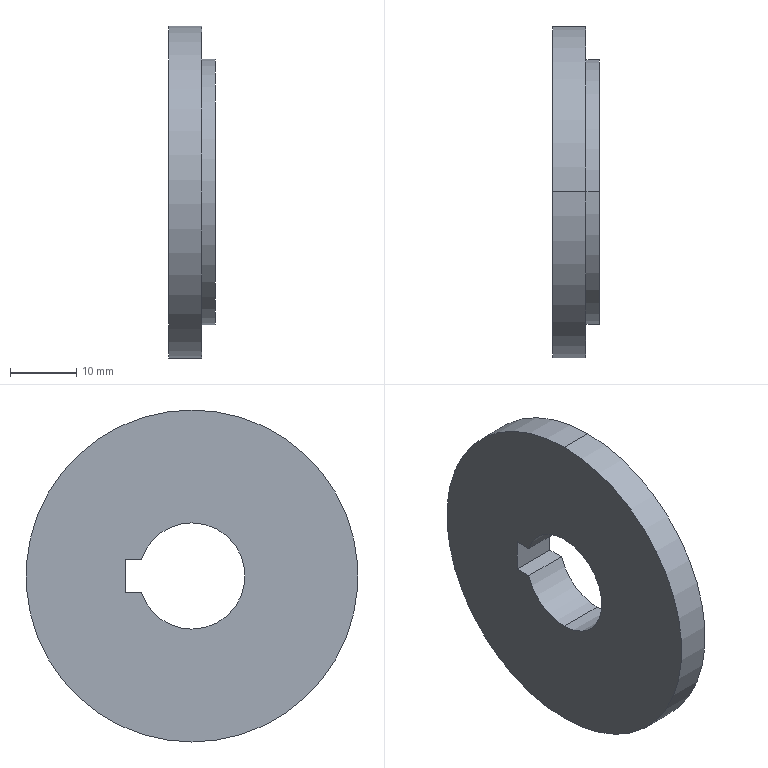Component | SolidWorks | MotorEndCover-1 | 1 solid | 13 faces | box 7 x 50 x 50 mm | volume 10847 mm3 | cylinder 7 | plane 6 | commonest cylinder face diameters 16 x3 50 x2 40 x2
build123d program:
from build123d import *

# Parameters (mm, degrees)
SKETCH2_R               = 20
BOSS_EXTRUDE1_DEPTH     = 2
SKETCH3_R               = 25
BOSS_EXTRUDE2_DEPTH     = 5
CUT_EXTRUDE1_DEPTH      = 37.042
CUT_EXTRUDE1_DEPTH_BACK = 37.042


with BuildPart() as part:
    # Sketch2 → Boss-Extrude1 (new body)
    with BuildSketch(Plane.XY):
        Circle(SKETCH2_R)
    extrude(amount=BOSS_EXTRUDE1_DEPTH)

    # Sketch3 → Boss-Extrude2 (add)
    with BuildSketch(Plane.XY.offset(2)):
        Circle(SKETCH3_R)
    extrude(amount=BOSS_EXTRUDE2_DEPTH)

    # Sketch4 → Cut-Extrude1 (cut, two sides: drawn at the far end of the back side and taken through both)
    with BuildSketch(Plane.XY.offset(7).offset(-CUT_EXTRUDE1_DEPTH_BACK)):
        with BuildLine():
            Line((-2.499, 7.6), (-2.499, 10.061))
            Line((-2.499, 10.061), (2.501, 10.061))
            Line((2.501, 10.061), (2.501, 7.599))
            ThreePointArc((2.501, 7.599), (-0.001053, -8), (-2.499, 7.6))
        make_face()
    extrude(amount=CUT_EXTRUDE1_DEPTH + CUT_EXTRUDE1_DEPTH_BACK, mode=Mode.SUBTRACT)


solid = part.part

# Placed as in the assembly
solid = solid.moved(Location((386.19, 335.1, 35), (0, -90, 0)))
STEP:
#1=COLOUR_RGB('',0.7922,0.8196,0.9333);
#2=FILL_AREA_STYLE_COLOUR('',#1);
#3=FILL_AREA_STYLE('',(#2));
#4=SURFACE_STYLE_FILL_AREA(#3);
#5=SURFACE_SIDE_STYLE('',(#4));
#6=SURFACE_STYLE_USAGE(.BOTH.,#5);
#7=PRESENTATION_STYLE_ASSIGNMENT((#6));
#8=CARTESIAN_POINT('',(15.204,13.193,1.063));
#9=VERTEX_POINT('',#8);
#10=CARTESIAN_POINT('',(15.204,13.193,1.693));
#11=VERTEX_POINT('',#10);
#12=CARTESIAN_POINT('',(15.204,13.193,1.378));
#13=DIRECTION('',(-1.,-0.,0.));
#14=DIRECTION('',(0.,-0.,1.));
#15=AXIS2_PLACEMENT_3D('',#12,#13,#14);
#16=CIRCLE('',#15,0.315);
#17=EDGE_CURVE('',#9,#11,#16,.T.);
#18=ORIENTED_EDGE('',*,*,#17,.F.);
#19=CARTESIAN_POINT('',(14.929,13.193,1.063));
#20=VERTEX_POINT('',#19);
#21=CARTESIAN_POINT('',(15.204,13.193,1.063));
#22=DIRECTION('',(-1.,-0.,0.));
#23=VECTOR('',#22,39.37);
#24=LINE('',#21,#23);
#25=EDGE_CURVE('',#9,#20,#24,.T.);
#26=ORIENTED_EDGE('',*,*,#25,.T.);
#27=CARTESIAN_POINT('',(14.929,13.193,1.693));
#28=VERTEX_POINT('',#27);
#29=CARTESIAN_POINT('',(14.929,13.193,1.378));
#30=DIRECTION('',(-1.,-0.,0.));
#31=DIRECTION('',(0.,-0.,1.));
#32=AXIS2_PLACEMENT_3D('',#29,#30,#31);
#33=CIRCLE('',#32,0.315);
#34=EDGE_CURVE('',#20,#28,#33,.T.);
#35=ORIENTED_EDGE('',*,*,#34,.T.);
#36=CARTESIAN_POINT('',(15.204,13.193,1.693));
#37=DIRECTION('',(-1.,-0.,0.));
#38=VECTOR('',#37,39.37);
#39=LINE('',#36,#38);
#40=EDGE_CURVE('',#11,#28,#39,.T.);
#41=ORIENTED_EDGE('',*,*,#40,.F.);
#42=EDGE_LOOP('',(#18,#26,#35,#41));
#43=FACE_OUTER_BOUND('',#42,.T.);
#44=CARTESIAN_POINT('',(15.204,13.193,1.378));
#45=DIRECTION('',(-1.,-0.,0.));
#46=DIRECTION('',(0.,-0.,1.));
#47=AXIS2_PLACEMENT_3D('',#44,#45,#46);
#48=CYLINDRICAL_SURFACE('',#47,0.315);
#49=ADVANCED_FACE('',(#43),#48,.F.);
#50=CARTESIAN_POINT('',(15.204,13.492,1.476));
#51=VERTEX_POINT('',#50);
#52=CARTESIAN_POINT('',(15.204,13.193,1.378));
#53=DIRECTION('',(-1.,-0.,0.));
#54=DIRECTION('',(0.,-0.,1.));
#55=AXIS2_PLACEMENT_3D('',#52,#53,#54);
#56=CIRCLE('',#55,0.315);
#57=EDGE_CURVE('',#11,#51,#56,.T.);
#58=ORIENTED_EDGE('',*,*,#57,.F.);
#59=ORIENTED_EDGE('',*,*,#40,.T.);
#60=CARTESIAN_POINT('',(14.929,13.492,1.476));
#61=VERTEX_POINT('',#60);
#62=CARTESIAN_POINT('',(14.929,13.193,1.378));
#63=DIRECTION('',(-1.,-0.,0.));
#64=DIRECTION('',(0.,-0.,1.));
#65=AXIS2_PLACEMENT_3D('',#62,#63,#64);
#66=CIRCLE('',#65,0.315);
#67=EDGE_CURVE('',#28,#61,#66,.T.);
#68=ORIENTED_EDGE('',*,*,#67,.T.);
#69=CARTESIAN_POINT('',(15.204,13.492,1.476));
#70=DIRECTION('',(-1.,-0.,0.));
#71=VECTOR('',#70,39.37);
#72=LINE('',#69,#71);
#73=EDGE_CURVE('',#51,#61,#72,.T.);
#74=ORIENTED_EDGE('',*,*,#73,.F.);
#75=EDGE_LOOP('',(#58,#59,#68,#74));
#76=FACE_OUTER_BOUND('',#75,.T.);
#77=CARTESIAN_POINT('',(15.204,13.193,1.378));
#78=DIRECTION('',(-1.,-0.,0.));
#79=DIRECTION('',(0.,-0.,1.));
#80=AXIS2_PLACEMENT_3D('',#77,#78,#79);
#81=CYLINDRICAL_SURFACE('',#80,0.315);
#82=ADVANCED_FACE('',(#76),#81,.F.);
#83=CARTESIAN_POINT('',(14.929,13.193,2.362));
#84=VERTEX_POINT('',#83);
#85=CARTESIAN_POINT('',(14.929,13.193,0.3937));
#86=VERTEX_POINT('',#85);
#87=CARTESIAN_POINT('',(14.929,13.193,1.378));
#88=DIRECTION('',(-1.,-0.,0.));
#89=DIRECTION('',(0.,-0.,1.));
#90=AXIS2_PLACEMENT_3D('',#87,#88,#89);
#91=CIRCLE('',#90,0.9843);
#92=EDGE_CURVE('',#84,#86,#91,.T.);
#93=ORIENTED_EDGE('',*,*,#92,.F.);
#94=CARTESIAN_POINT('',(15.126,13.193,2.362));
#95=VERTEX_POINT('',#94);
#96=CARTESIAN_POINT('',(14.929,13.193,2.362));
#97=DIRECTION('',(1.,0.,-0.));
#98=VECTOR('',#97,39.37);
#99=LINE('',#96,#98);
#100=EDGE_CURVE('',#84,#95,#99,.T.);
#101=ORIENTED_EDGE('',*,*,#100,.T.);
#102=CARTESIAN_POINT('',(15.126,13.193,0.3937));
#103=VERTEX_POINT('',#102);
#104=CARTESIAN_POINT('',(15.126,13.193,1.378));
#105=DIRECTION('',(-1.,-0.,0.));
#106=DIRECTION('',(0.,-0.,1.));
#107=AXIS2_PLACEMENT_3D('',#104,#105,#106);
#108=CIRCLE('',#107,0.9843);
#109=EDGE_CURVE('',#95,#103,#108,.T.);
#110=ORIENTED_EDGE('',*,*,#109,.T.);
#111=CARTESIAN_POINT('',(14.929,13.193,0.3937));
#112=DIRECTION('',(1.,0.,-0.));
#113=VECTOR('',#112,39.37);
#114=LINE('',#111,#113);
#115=EDGE_CURVE('',#86,#103,#114,.T.);
#116=ORIENTED_EDGE('',*,*,#115,.F.);
#117=EDGE_LOOP('',(#93,#101,#110,#116));
#118=FACE_OUTER_BOUND('',#117,.T.);
#119=CARTESIAN_POINT('',(14.929,13.193,1.378));
#120=DIRECTION('',(1.,0.,-0.));
#121=DIRECTION('',(0.,0.,-1.));
#122=AXIS2_PLACEMENT_3D('',#119,#120,#121);
#123=CYLINDRICAL_SURFACE('',#122,0.9843);
#124=ADVANCED_FACE('',(#118),#123,.T.);
#125=CARTESIAN_POINT('',(15.126,13.193,2.165));
#126=VERTEX_POINT('',#125);
#127=CARTESIAN_POINT('',(15.126,13.193,0.5906));
#128=VERTEX_POINT('',#127);
#129=CARTESIAN_POINT('',(15.126,13.193,1.378));
#130=DIRECTION('',(-1.,-0.,0.));
#131=DIRECTION('',(0.,-0.,1.));
#132=AXIS2_PLACEMENT_3D('',#129,#130,#131);
#133=CIRCLE('',#132,0.7874);
#134=EDGE_CURVE('',#126,#128,#133,.T.);
#135=ORIENTED_EDGE('',*,*,#134,.F.);
#136=CARTESIAN_POINT('',(15.204,13.193,2.165));
#137=VERTEX_POINT('',#136);
#138=CARTESIAN_POINT('',(15.126,13.193,2.165));
#139=DIRECTION('',(1.,0.,-0.));
#140=VECTOR('',#139,39.37);
#141=LINE('',#138,#140);
#142=EDGE_CURVE('',#126,#137,#141,.T.);
#143=ORIENTED_EDGE('',*,*,#142,.T.);
#144=CARTESIAN_POINT('',(15.204,13.193,0.5906));
#145=VERTEX_POINT('',#144);
#146=CARTESIAN_POINT('',(15.204,13.193,1.378));
#147=DIRECTION('',(-1.,-0.,0.));
#148=DIRECTION('',(0.,-0.,1.));
#149=AXIS2_PLACEMENT_3D('',#146,#147,#148);
#150=CIRCLE('',#149,0.7874);
#151=EDGE_CURVE('',#137,#145,#150,.T.);
#152=ORIENTED_EDGE('',*,*,#151,.T.);
#153=CARTESIAN_POINT('',(15.126,13.193,0.5906));
#154=DIRECTION('',(1.,0.,-0.));
#155=VECTOR('',#154,39.37);
#156=LINE('',#153,#155);
#157=EDGE_CURVE('',#128,#145,#156,.T.);
#158=ORIENTED_EDGE('',*,*,#157,.F.);
#159=EDGE_LOOP('',(#135,#143,#152,#158));
#160=FACE_OUTER_BOUND('',#159,.T.);
#161=CARTESIAN_POINT('',(15.126,13.193,1.378));
#162=DIRECTION('',(1.,0.,-0.));
#163=DIRECTION('',(0.,0.,-1.));
#164=AXIS2_PLACEMENT_3D('',#161,#162,#163);
#165=CYLINDRICAL_SURFACE('',#164,0.7874);
#166=ADVANCED_FACE('',(#160),#165,.T.);
#167=CARTESIAN_POINT('',(15.204,13.193,1.378));
#168=DIRECTION('',(-1.,-0.,0.));
#169=DIRECTION('',(0.,-0.,1.));
#170=AXIS2_PLACEMENT_3D('',#167,#168,#169);
#171=CIRCLE('',#170,0.7874);
#172=EDGE_CURVE('',#145,#137,#171,.T.);
#173=ORIENTED_EDGE('',*,*,#172,.F.);
#174=ORIENTED_EDGE('',*,*,#151,.F.);
#175=EDGE_LOOP('',(#173,#174));
#176=FACE_OUTER_BOUND('',#175,.T.);
#177=CARTESIAN_POINT('',(15.204,13.589,1.476));
#178=VERTEX_POINT('',#177);
#179=CARTESIAN_POINT('',(15.204,13.589,1.476));
#180=DIRECTION('',(-0.,1.,0.));
#181=VECTOR('',#180,39.37);
#182=LINE('',#179,#181);
#183=EDGE_CURVE('',#51,#178,#182,.T.);
#184=ORIENTED_EDGE('',*,*,#183,.T.);
#185=CARTESIAN_POINT('',(15.204,13.589,1.28));
#186=VERTEX_POINT('',#185);
#187=CARTESIAN_POINT('',(15.204,13.589,1.28));
#188=DIRECTION('',(-0.,0.,-1.));
#189=VECTOR('',#188,39.37);
#190=LINE('',#187,#189);
#191=EDGE_CURVE('',#178,#186,#190,.T.);
#192=ORIENTED_EDGE('',*,*,#191,.T.);
#193=CARTESIAN_POINT('',(15.204,13.492,1.28));
#194=VERTEX_POINT('',#193);
#195=CARTESIAN_POINT('',(15.204,13.492,1.28));
#196=DIRECTION('',(0.,-1.,-0.));
#197=VECTOR('',#196,39.37);
#198=LINE('',#195,#197);
#199=EDGE_CURVE('',#186,#194,#198,.T.);
#200=ORIENTED_EDGE('',*,*,#199,.T.);
#201=CARTESIAN_POINT('',(15.204,13.193,1.378));
#202=DIRECTION('',(-1.,-0.,0.));
#203=DIRECTION('',(0.,-0.,1.));
#204=AXIS2_PLACEMENT_3D('',#201,#202,#203);
#205=CIRCLE('',#204,0.315);
#206=EDGE_CURVE('',#194,#9,#205,.T.);
#207=ORIENTED_EDGE('',*,*,#206,.T.);
#208=ORIENTED_EDGE('',*,*,#17,.T.);
#209=ORIENTED_EDGE('',*,*,#57,.T.);
#210=EDGE_LOOP('',(#184,#192,#200,#207,#208,#209));
#211=FACE_BOUND('',#210,.T.);
#212=CARTESIAN_POINT('',(15.204,13.193,1.378));
#213=DIRECTION('',(-1.,-0.,0.));
#214=DIRECTION('',(0.,-0.,1.));
#215=AXIS2_PLACEMENT_3D('',#212,#213,#214);
#216=PLANE('',#215);
#217=ADVANCED_FACE('',(#176,#211),#216,.F.);
#218=CARTESIAN_POINT('',(14.929,13.193,1.378));
#219=DIRECTION('',(-1.,-0.,0.));
#220=DIRECTION('',(0.,-0.,1.));
#221=AXIS2_PLACEMENT_3D('',#218,#219,#220);
#222=CIRCLE('',#221,0.9843);
#223=EDGE_CURVE('',#86,#84,#222,.T.);
#224=ORIENTED_EDGE('',*,*,#223,.T.);
#225=ORIENTED_EDGE('',*,*,#92,.T.);
#226=EDGE_LOOP('',(#224,#225));
#227=FACE_OUTER_BOUND('',#226,.T.);
#228=CARTESIAN_POINT('',(14.929,13.589,1.28));
#229=VERTEX_POINT('',#228);
#230=CARTESIAN_POINT('',(14.929,13.589,1.476));
#231=VERTEX_POINT('',#230);
#232=CARTESIAN_POINT('',(14.929,13.589,1.378));
#233=DIRECTION('',(0.,-0.,1.));
#234=VECTOR('',#233,39.37);
#235=LINE('',#232,#234);
#236=EDGE_CURVE('',#229,#231,#235,.T.);
#237=ORIENTED_EDGE('',*,*,#236,.T.);
#238=CARTESIAN_POINT('',(14.929,13.193,1.476));
#239=DIRECTION('',(0.,-1.,-0.));
#240=VECTOR('',#239,39.37);
#241=LINE('',#238,#240);
#242=EDGE_CURVE('',#231,#61,#241,.T.);
#243=ORIENTED_EDGE('',*,*,#242,.T.);
#244=ORIENTED_EDGE('',*,*,#67,.F.);
#245=ORIENTED_EDGE('',*,*,#34,.F.);
#246=CARTESIAN_POINT('',(14.929,13.492,1.28));
#247=VERTEX_POINT('',#246);
#248=CARTESIAN_POINT('',(14.929,13.193,1.378));
#249=DIRECTION('',(-1.,-0.,0.));
#250=DIRECTION('',(0.,-0.,1.));
#251=AXIS2_PLACEMENT_3D('',#248,#249,#250);
#252=CIRCLE('',#251,0.315);
#253=EDGE_CURVE('',#247,#20,#252,.T.);
#254=ORIENTED_EDGE('',*,*,#253,.F.);
#255=CARTESIAN_POINT('',(14.929,13.193,1.28));
#256=DIRECTION('',(-0.,1.,0.));
#257=VECTOR('',#256,39.37);
#258=LINE('',#255,#257);
#259=EDGE_CURVE('',#247,#229,#258,.T.);
#260=ORIENTED_EDGE('',*,*,#259,.T.);
#261=EDGE_LOOP('',(#237,#243,#244,#245,#254,#260));
#262=FACE_BOUND('',#261,.T.);
#263=CARTESIAN_POINT('',(14.929,13.193,1.378));
#264=DIRECTION('',(-1.,-0.,0.));
#265=DIRECTION('',(0.,-0.,1.));
#266=AXIS2_PLACEMENT_3D('',#263,#264,#265);
#267=PLANE('',#266);
#268=ADVANCED_FACE('',(#227,#262),#267,.T.);
#269=ORIENTED_EDGE('',*,*,#142,.F.);
#270=CARTESIAN_POINT('',(15.126,13.193,1.378));
#271=DIRECTION('',(-1.,-0.,0.));
#272=DIRECTION('',(0.,-0.,1.));
#273=AXIS2_PLACEMENT_3D('',#270,#271,#272);
#274=CIRCLE('',#273,0.7874);
#275=EDGE_CURVE('',#128,#126,#274,.T.);
#276=ORIENTED_EDGE('',*,*,#275,.F.);
#277=ORIENTED_EDGE('',*,*,#157,.T.);
#278=ORIENTED_EDGE('',*,*,#172,.T.);
#279=EDGE_LOOP('',(#269,#276,#277,#278));
#280=FACE_OUTER_BOUND('',#279,.T.);
#281=CARTESIAN_POINT('',(15.126,13.193,1.378));
#282=DIRECTION('',(1.,0.,-0.));
#283=DIRECTION('',(0.,0.,-1.));
#284=AXIS2_PLACEMENT_3D('',#281,#282,#283);
#285=CYLINDRICAL_SURFACE('',#284,0.7874);
#286=ADVANCED_FACE('',(#280),#285,.T.);
#287=ORIENTED_EDGE('',*,*,#100,.F.);
#288=ORIENTED_EDGE('',*,*,#223,.F.);
#289=ORIENTED_EDGE('',*,*,#115,.T.);
#290=CARTESIAN_POINT('',(15.126,13.193,1.378));
#291=DIRECTION('',(-1.,-0.,0.));
#292=DIRECTION('',(0.,-0.,1.));
#293=AXIS2_PLACEMENT_3D('',#290,#291,#292);
#294=CIRCLE('',#293,0.9843);
#295=EDGE_CURVE('',#103,#95,#294,.T.);
#296=ORIENTED_EDGE('',*,*,#295,.T.);
#297=EDGE_LOOP('',(#287,#288,#289,#296));
#298=FACE_OUTER_BOUND('',#297,.T.);
#299=CARTESIAN_POINT('',(14.929,13.193,1.378));
#300=DIRECTION('',(1.,0.,-0.));
#301=DIRECTION('',(0.,0.,-1.));
#302=AXIS2_PLACEMENT_3D('',#299,#300,#301);
#303=CYLINDRICAL_SURFACE('',#302,0.9843);
#304=ADVANCED_FACE('',(#298),#303,.T.);
#305=ORIENTED_EDGE('',*,*,#275,.T.);
#306=ORIENTED_EDGE('',*,*,#134,.T.);
#307=EDGE_LOOP('',(#305,#306));
#308=FACE_BOUND('',#307,.T.);
#309=ORIENTED_EDGE('',*,*,#295,.F.);
#310=ORIENTED_EDGE('',*,*,#109,.F.);
#311=EDGE_LOOP('',(#309,#310));
#312=FACE_OUTER_BOUND('',#311,.T.);
#313=CARTESIAN_POINT('',(15.126,13.193,1.378));
#314=DIRECTION('',(-1.,-0.,0.));
#315=DIRECTION('',(0.,-0.,1.));
#316=AXIS2_PLACEMENT_3D('',#313,#314,#315);
#317=PLANE('',#316);
#318=ADVANCED_FACE('',(#308,#312),#317,.F.);
#319=CARTESIAN_POINT('',(14.929,13.589,1.476));
#320=DIRECTION('',(1.,0.,-0.));
#321=VECTOR('',#320,39.37);
#322=LINE('',#319,#321);
#323=EDGE_CURVE('',#231,#178,#322,.T.);
#324=ORIENTED_EDGE('',*,*,#323,.T.);
#325=ORIENTED_EDGE('',*,*,#183,.F.);
#326=ORIENTED_EDGE('',*,*,#73,.T.);
#327=ORIENTED_EDGE('',*,*,#242,.F.);
#328=EDGE_LOOP('',(#324,#325,#326,#327));
#329=FACE_OUTER_BOUND('',#328,.T.);
#330=CARTESIAN_POINT('',(14.929,13.589,1.476));
#331=DIRECTION('',(-0.,0.,-1.));
#332=DIRECTION('',(0.,-1.,-0.));
#333=AXIS2_PLACEMENT_3D('',#330,#331,#332);
#334=PLANE('',#333);
#335=ADVANCED_FACE('',(#329),#334,.T.);
#336=CARTESIAN_POINT('',(14.929,13.589,1.28));
#337=DIRECTION('',(1.,0.,-0.));
#338=VECTOR('',#337,39.37);
#339=LINE('',#336,#338);
#340=EDGE_CURVE('',#229,#186,#339,.T.);
#341=ORIENTED_EDGE('',*,*,#340,.T.);
#342=ORIENTED_EDGE('',*,*,#191,.F.);
#343=ORIENTED_EDGE('',*,*,#323,.F.);
#344=ORIENTED_EDGE('',*,*,#236,.F.);
#345=EDGE_LOOP('',(#341,#342,#343,#344));
#346=FACE_OUTER_BOUND('',#345,.T.);
#347=CARTESIAN_POINT('',(14.929,13.589,1.28));
#348=DIRECTION('',(0.,-1.,-0.));
#349=DIRECTION('',(1.,0.,-0.));
#350=AXIS2_PLACEMENT_3D('',#347,#348,#349);
#351=PLANE('',#350);
#352=ADVANCED_FACE('',(#346),#351,.T.);
#353=CARTESIAN_POINT('',(15.204,13.492,1.28));
#354=DIRECTION('',(-1.,-0.,0.));
#355=VECTOR('',#354,39.37);
#356=LINE('',#353,#355);
#357=EDGE_CURVE('',#194,#247,#356,.T.);
#358=ORIENTED_EDGE('',*,*,#357,.F.);
#359=ORIENTED_EDGE('',*,*,#199,.F.);
#360=ORIENTED_EDGE('',*,*,#340,.F.);
#361=ORIENTED_EDGE('',*,*,#259,.F.);
#362=EDGE_LOOP('',(#358,#359,#360,#361));
#363=FACE_OUTER_BOUND('',#362,.T.);
#364=CARTESIAN_POINT('',(14.929,13.492,1.28));
#365=DIRECTION('',(0.,-0.,1.));
#366=DIRECTION('',(-0.,1.,0.));
#367=AXIS2_PLACEMENT_3D('',#364,#365,#366);
#368=PLANE('',#367);
#369=ADVANCED_FACE('',(#363),#368,.T.);
#370=ORIENTED_EDGE('',*,*,#25,.F.);
#371=ORIENTED_EDGE('',*,*,#206,.F.);
#372=ORIENTED_EDGE('',*,*,#357,.T.);
#373=ORIENTED_EDGE('',*,*,#253,.T.);
#374=EDGE_LOOP('',(#370,#371,#372,#373));
#375=FACE_OUTER_BOUND('',#374,.T.);
#376=CARTESIAN_POINT('',(15.204,13.193,1.378));
#377=DIRECTION('',(-1.,-0.,0.));
#378=DIRECTION('',(0.,-0.,1.));
#379=AXIS2_PLACEMENT_3D('',#376,#377,#378);
#380=CYLINDRICAL_SURFACE('',#379,0.315);
#381=ADVANCED_FACE('',(#375),#380,.F.);
#382=CLOSED_SHELL('',(#49,#82,#124,#166,#217,#268,#286,#304,#318,#335,#352,#369,#381));
#383=MANIFOLD_SOLID_BREP('',#382);
#384=STYLED_ITEM('',(#7),#383);
#385=(LENGTH_UNIT()NAMED_UNIT(*)SI_UNIT($,.METRE.));
#386=LENGTH_MEASURE_WITH_UNIT(LENGTH_MEASURE(0.0254),#385);
#387=DIMENSIONAL_EXPONENTS(1.,0.,0.,0.,0.,0.,0.);
#388=(CONVERSION_BASED_UNIT('',#386)LENGTH_UNIT()NAMED_UNIT(#387));
#389=UNCERTAINTY_MEASURE_WITH_UNIT(LENGTH_MEASURE(0.00001),#388,'','');
#390=(NAMED_UNIT(*)PLANE_ANGLE_UNIT()SI_UNIT($,.RADIAN.));
#391=(NAMED_UNIT(*)SI_UNIT($,.STERADIAN.)SOLID_ANGLE_UNIT());
#392=(GEOMETRIC_REPRESENTATION_CONTEXT(3)GLOBAL_UNCERTAINTY_ASSIGNED_CONTEXT((#389))GLOBAL_UNIT_ASSIGNED_CONTEXT((#388,#390,#391))REPRESENTATION_CONTEXT('',''));
#393=MECHANICAL_DESIGN_GEOMETRIC_PRESENTATION_REPRESENTATION('',(#384),#392);
#394=PRESENTATION_LAYER_ASSIGNMENT('','',(#384));
#395=CARTESIAN_POINT('',(0.,0.,0.));
#396=DIRECTION('',(0.,0.,1.));
#397=DIRECTION('',(1.,0.,0.));
#398=AXIS2_PLACEMENT_3D('',#395,#396,#397);
#399=(LENGTH_UNIT()NAMED_UNIT(*)SI_UNIT($,.METRE.));
#400=LENGTH_MEASURE_WITH_UNIT(LENGTH_MEASURE(0.0254),#399);
#401=DIMENSIONAL_EXPONENTS(1.,0.,0.,0.,0.,0.,0.);
#402=(CONVERSION_BASED_UNIT('',#400)LENGTH_UNIT()NAMED_UNIT(#401));
#403=UNCERTAINTY_MEASURE_WITH_UNIT(LENGTH_MEASURE(0.00001),#402,'','');
#404=(NAMED_UNIT(*)PLANE_ANGLE_UNIT()SI_UNIT($,.RADIAN.));
#405=(NAMED_UNIT(*)SI_UNIT($,.STERADIAN.)SOLID_ANGLE_UNIT());
#406=(GEOMETRIC_REPRESENTATION_CONTEXT(3)GLOBAL_UNCERTAINTY_ASSIGNED_CONTEXT((#403))GLOBAL_UNIT_ASSIGNED_CONTEXT((#402,#404,#405))REPRESENTATION_CONTEXT('',''));
#407=ADVANCED_BREP_SHAPE_REPRESENTATION('',(#383,#398),#406);